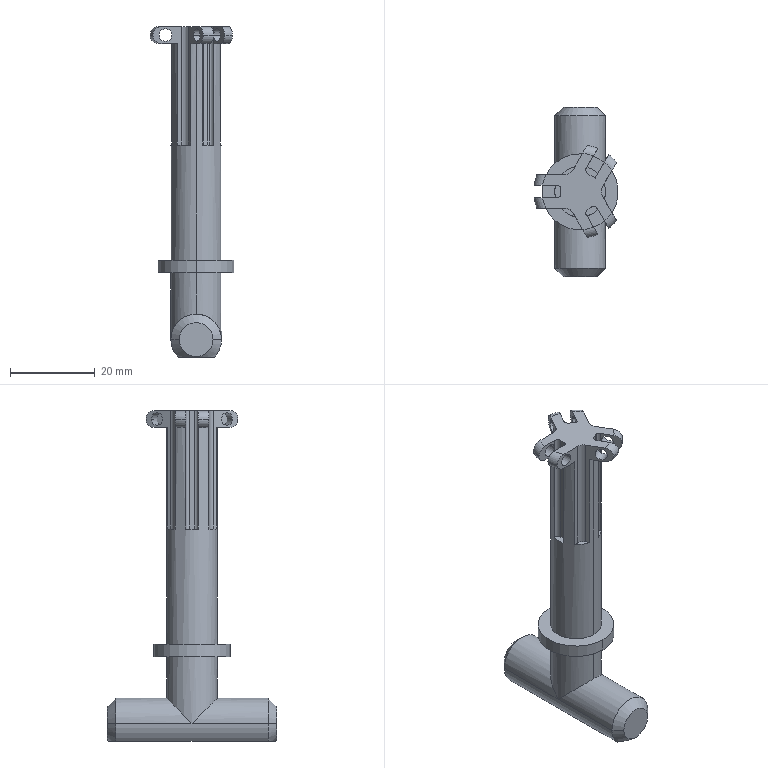Component | SolidWorks | g-1 | 1 solid | 82 faces | volume 11853 mm3 | cylinder 33 | plane 33 | torus 12 | cone 4 | commonest cylinder face diameters 3 x12 2 x8 12 x8 4 x3 18 x2